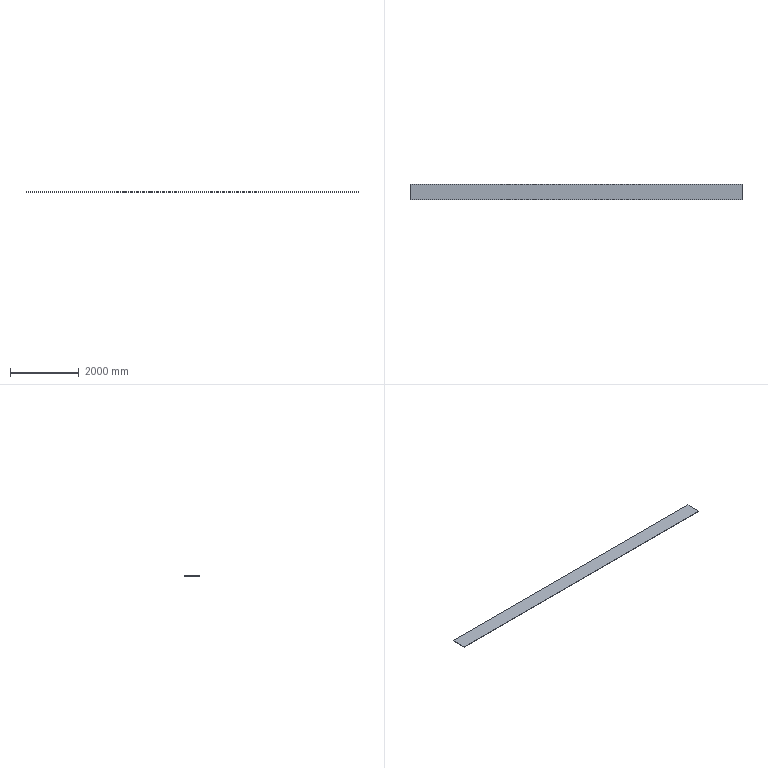Component | SolidWorks | Main-1_9940X450X10-1 | 1 solid | 6 faces | box 9670 x 450 x 10 mm | volume 43515000 mm3 | plane 6 | material Plain Carbon Steel
STEP:
#1=CARTESIAN_POINT('',(-132.764,84.501,219.527));
#2=VERTEX_POINT('',#1);
#3=CARTESIAN_POINT('',(-132.764,66.784,219.527));
#4=VERTEX_POINT('',#3);
#5=CARTESIAN_POINT('',(-132.764,84.501,219.527));
#6=DIRECTION('',(0.,-1.,-0.));
#7=VECTOR('',#6,39.37);
#8=LINE('',#5,#7);
#9=EDGE_CURVE('',#2,#4,#8,.T.);
#10=ORIENTED_EDGE('',*,*,#9,.F.);
#11=CARTESIAN_POINT('',(-132.764,84.501,219.133));
#12=VERTEX_POINT('',#11);
#13=CARTESIAN_POINT('',(-132.764,84.501,219.133));
#14=DIRECTION('',(0.,-0.,1.));
#15=VECTOR('',#14,39.37);
#16=LINE('',#13,#15);
#17=EDGE_CURVE('',#12,#2,#16,.T.);
#18=ORIENTED_EDGE('',*,*,#17,.F.);
#19=CARTESIAN_POINT('',(-132.764,66.784,219.133));
#20=VERTEX_POINT('',#19);
#21=CARTESIAN_POINT('',(-132.764,84.501,219.133));
#22=DIRECTION('',(0.,-1.,-0.));
#23=VECTOR('',#22,39.37);
#24=LINE('',#21,#23);
#25=EDGE_CURVE('',#12,#20,#24,.T.);
#26=ORIENTED_EDGE('',*,*,#25,.T.);
#27=CARTESIAN_POINT('',(-132.764,66.784,219.133));
#28=DIRECTION('',(0.,-0.,1.));
#29=VECTOR('',#28,39.37);
#30=LINE('',#27,#29);
#31=EDGE_CURVE('',#20,#4,#30,.T.);
#32=ORIENTED_EDGE('',*,*,#31,.T.);
#33=EDGE_LOOP('',(#10,#18,#26,#32));
#34=FACE_OUTER_BOUND('',#33,.T.);
#35=CARTESIAN_POINT('',(-132.764,84.501,219.133));
#36=DIRECTION('',(-1.,-0.,-0.));
#37=DIRECTION('',(0.,-1.,-0.));
#38=AXIS2_PLACEMENT_3D('',#35,#36,#37);
#39=PLANE('',#38);
#40=ADVANCED_FACE('',(#34),#39,.T.);
#41=CARTESIAN_POINT('',(247.945,84.501,219.527));
#42=VERTEX_POINT('',#41);
#43=CARTESIAN_POINT('',(-132.764,84.501,219.527));
#44=DIRECTION('',(-1.,0.,0.));
#45=VECTOR('',#44,39.37);
#46=LINE('',#43,#45);
#47=EDGE_CURVE('',#42,#2,#46,.T.);
#48=ORIENTED_EDGE('',*,*,#47,.F.);
#49=CARTESIAN_POINT('',(247.945,84.501,219.133));
#50=VERTEX_POINT('',#49);
#51=CARTESIAN_POINT('',(247.945,84.501,219.133));
#52=DIRECTION('',(0.,-0.,1.));
#53=VECTOR('',#52,39.37);
#54=LINE('',#51,#53);
#55=EDGE_CURVE('',#50,#42,#54,.T.);
#56=ORIENTED_EDGE('',*,*,#55,.F.);
#57=CARTESIAN_POINT('',(-132.764,84.501,219.133));
#58=DIRECTION('',(-1.,0.,0.));
#59=VECTOR('',#58,39.37);
#60=LINE('',#57,#59);
#61=EDGE_CURVE('',#50,#12,#60,.T.);
#62=ORIENTED_EDGE('',*,*,#61,.T.);
#63=ORIENTED_EDGE('',*,*,#17,.T.);
#64=EDGE_LOOP('',(#48,#56,#62,#63));
#65=FACE_OUTER_BOUND('',#64,.T.);
#66=CARTESIAN_POINT('',(-132.764,84.501,219.133));
#67=DIRECTION('',(0.,1.,0.));
#68=DIRECTION('',(-1.,0.,0.));
#69=AXIS2_PLACEMENT_3D('',#66,#67,#68);
#70=PLANE('',#69);
#71=ADVANCED_FACE('',(#65),#70,.T.);
#72=CARTESIAN_POINT('',(247.945,66.784,219.527));
#73=VERTEX_POINT('',#72);
#74=CARTESIAN_POINT('',(247.945,84.501,219.527));
#75=DIRECTION('',(0.,1.,0.));
#76=VECTOR('',#75,39.37);
#77=LINE('',#74,#76);
#78=EDGE_CURVE('',#73,#42,#77,.T.);
#79=ORIENTED_EDGE('',*,*,#78,.F.);
#80=CARTESIAN_POINT('',(247.945,66.784,219.133));
#81=VERTEX_POINT('',#80);
#82=CARTESIAN_POINT('',(247.945,66.784,219.133));
#83=DIRECTION('',(0.,-0.,1.));
#84=VECTOR('',#83,39.37);
#85=LINE('',#82,#84);
#86=EDGE_CURVE('',#81,#73,#85,.T.);
#87=ORIENTED_EDGE('',*,*,#86,.F.);
#88=CARTESIAN_POINT('',(247.945,84.501,219.133));
#89=DIRECTION('',(0.,1.,0.));
#90=VECTOR('',#89,39.37);
#91=LINE('',#88,#90);
#92=EDGE_CURVE('',#81,#50,#91,.T.);
#93=ORIENTED_EDGE('',*,*,#92,.T.);
#94=ORIENTED_EDGE('',*,*,#55,.T.);
#95=EDGE_LOOP('',(#79,#87,#93,#94));
#96=FACE_OUTER_BOUND('',#95,.T.);
#97=CARTESIAN_POINT('',(247.945,84.501,219.133));
#98=DIRECTION('',(1.,0.,0.));
#99=DIRECTION('',(0.,1.,0.));
#100=AXIS2_PLACEMENT_3D('',#97,#98,#99);
#101=PLANE('',#100);
#102=ADVANCED_FACE('',(#96),#101,.T.);
#103=CARTESIAN_POINT('',(-132.764,66.784,219.527));
#104=DIRECTION('',(1.,0.,0.));
#105=VECTOR('',#104,39.37);
#106=LINE('',#103,#105);
#107=EDGE_CURVE('',#4,#73,#106,.T.);
#108=ORIENTED_EDGE('',*,*,#107,.F.);
#109=ORIENTED_EDGE('',*,*,#31,.F.);
#110=CARTESIAN_POINT('',(-132.764,66.784,219.133));
#111=DIRECTION('',(1.,0.,0.));
#112=VECTOR('',#111,39.37);
#113=LINE('',#110,#112);
#114=EDGE_CURVE('',#20,#81,#113,.T.);
#115=ORIENTED_EDGE('',*,*,#114,.T.);
#116=ORIENTED_EDGE('',*,*,#86,.T.);
#117=EDGE_LOOP('',(#108,#109,#115,#116));
#118=FACE_OUTER_BOUND('',#117,.T.);
#119=CARTESIAN_POINT('',(-132.764,66.784,219.133));
#120=DIRECTION('',(0.,-1.,-0.));
#121=DIRECTION('',(1.,0.,0.));
#122=AXIS2_PLACEMENT_3D('',#119,#120,#121);
#123=PLANE('',#122);
#124=ADVANCED_FACE('',(#118),#123,.T.);
#125=ORIENTED_EDGE('',*,*,#25,.F.);
#126=ORIENTED_EDGE('',*,*,#61,.F.);
#127=ORIENTED_EDGE('',*,*,#92,.F.);
#128=ORIENTED_EDGE('',*,*,#114,.F.);
#129=EDGE_LOOP('',(#125,#126,#127,#128));
#130=FACE_OUTER_BOUND('',#129,.T.);
#131=CARTESIAN_POINT('',(-132.764,84.501,219.133));
#132=DIRECTION('',(0.,-0.,1.));
#133=DIRECTION('',(0.,-1.,-0.));
#134=AXIS2_PLACEMENT_3D('',#131,#132,#133);
#135=PLANE('',#134);
#136=ADVANCED_FACE('',(#130),#135,.F.);
#137=ORIENTED_EDGE('',*,*,#9,.T.);
#138=ORIENTED_EDGE('',*,*,#107,.T.);
#139=ORIENTED_EDGE('',*,*,#78,.T.);
#140=ORIENTED_EDGE('',*,*,#47,.T.);
#141=EDGE_LOOP('',(#137,#138,#139,#140));
#142=FACE_OUTER_BOUND('',#141,.T.);
#143=CARTESIAN_POINT('',(-132.764,84.501,219.527));
#144=DIRECTION('',(0.,-0.,1.));
#145=DIRECTION('',(0.,-1.,-0.));
#146=AXIS2_PLACEMENT_3D('',#143,#144,#145);
#147=PLANE('',#146);
#148=ADVANCED_FACE('',(#142),#147,.T.);
#149=CLOSED_SHELL('',(#40,#71,#102,#124,#136,#148));
#150=MANIFOLD_SOLID_BREP('',#149);
#151=CARTESIAN_POINT('',(0.,0.,0.));
#152=DIRECTION('',(0.,0.,1.));
#153=DIRECTION('',(1.,0.,0.));
#154=AXIS2_PLACEMENT_3D('',#151,#152,#153);
#155=(LENGTH_UNIT()NAMED_UNIT(*)SI_UNIT($,.METRE.));
#156=LENGTH_MEASURE_WITH_UNIT(LENGTH_MEASURE(0.0254),#155);
#157=DIMENSIONAL_EXPONENTS(1.,0.,0.,0.,0.,0.,0.);
#158=(CONVERSION_BASED_UNIT('',#156)LENGTH_UNIT()NAMED_UNIT(#157));
#159=UNCERTAINTY_MEASURE_WITH_UNIT(LENGTH_MEASURE(0.00001),#158,'','');
#160=(NAMED_UNIT(*)PLANE_ANGLE_UNIT()SI_UNIT($,.RADIAN.));
#161=(NAMED_UNIT(*)SI_UNIT($,.STERADIAN.)SOLID_ANGLE_UNIT());
#162=(GEOMETRIC_REPRESENTATION_CONTEXT(3)GLOBAL_UNCERTAINTY_ASSIGNED_CONTEXT((#159))GLOBAL_UNIT_ASSIGNED_CONTEXT((#158,#160,#161))REPRESENTATION_CONTEXT('',''));
#163=ADVANCED_BREP_SHAPE_REPRESENTATION('',(#150,#154),#162);
#164=COLOUR_RGB('',0.7922,0.8196,0.9333);
#165=FILL_AREA_STYLE_COLOUR('',#164);
#166=FILL_AREA_STYLE('',(#165));
#167=SURFACE_STYLE_FILL_AREA(#166);
#168=SURFACE_SIDE_STYLE('',(#167));
#169=SURFACE_STYLE_USAGE(.BOTH.,#168);
#170=PRESENTATION_STYLE_ASSIGNMENT((#169));
#171=STYLED_ITEM('',(#170),#150);
#172=(LENGTH_UNIT()NAMED_UNIT(*)SI_UNIT($,.METRE.));
#173=LENGTH_MEASURE_WITH_UNIT(LENGTH_MEASURE(0.0254),#172);
#174=DIMENSIONAL_EXPONENTS(1.,0.,0.,0.,0.,0.,0.);
#175=(CONVERSION_BASED_UNIT('',#173)LENGTH_UNIT()NAMED_UNIT(#174));
#176=UNCERTAINTY_MEASURE_WITH_UNIT(LENGTH_MEASURE(0.00001),#175,'','');
#177=(NAMED_UNIT(*)PLANE_ANGLE_UNIT()SI_UNIT($,.RADIAN.));
#178=(NAMED_UNIT(*)SI_UNIT($,.STERADIAN.)SOLID_ANGLE_UNIT());
#179=(GEOMETRIC_REPRESENTATION_CONTEXT(3)GLOBAL_UNCERTAINTY_ASSIGNED_CONTEXT((#176))GLOBAL_UNIT_ASSIGNED_CONTEXT((#175,#177,#178))REPRESENTATION_CONTEXT('',''));
#180=MECHANICAL_DESIGN_GEOMETRIC_PRESENTATION_REPRESENTATION('',(#171),#179);
#181=PRESENTATION_LAYER_ASSIGNMENT('','',(#171));